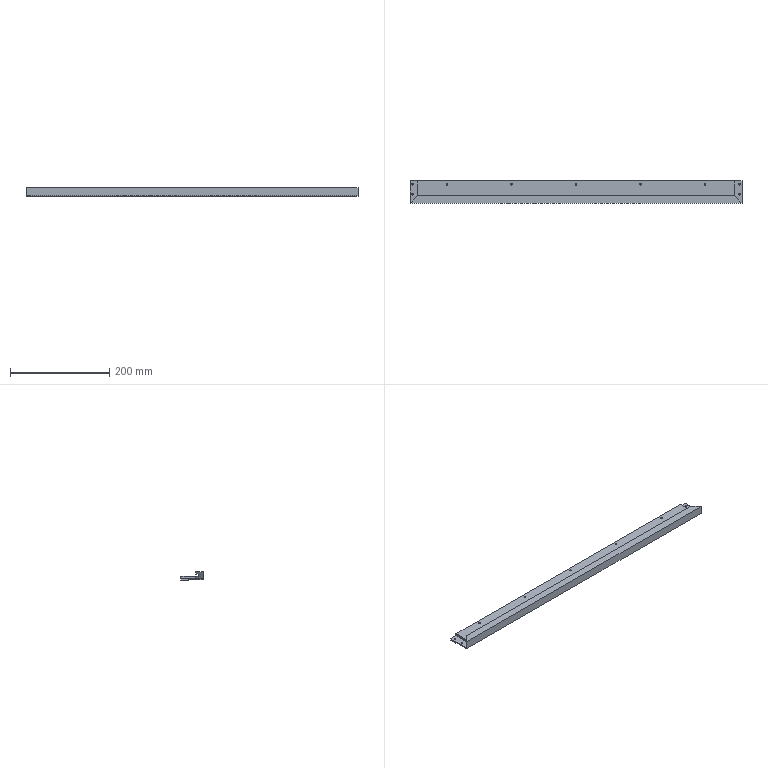Component | SolidWorks | AUTO-SpinDryWashing-01-03000004-1 | 1 solid | 36 faces | box 670 x 45 x 18 mm | volume 297172 mm3 | cylinder 18 | plane 18 | commonest cylinder face diameters 3.3 x18 | material AISI 316 Stainless Steel Sheet (SS)
build123d program:
from build123d import *

# Parameters (mm, degrees)
SKETCH1_W           = 20
SKETCH1_H           = 15
BOSS_EXTRUDE1_DEPTH = 335
SKETCH2_W           = 15
SKETCH2_H           = 30
BOSS_EXTRUDE2_DEPTH = 335
CUT_EXTRUDE2_DEPTH  = 671.746
CUT_EXTRUDE3_DEPTH  = 13
M4_TAPPED_HOLE1_D   = 3.3
M4_TAPPED_HOLE2_D   = 3.3
BOSS_EXTRUDE3_DEPTH = 2
SKETCH11_W          = 4
SKETCH11_H          = 15
CUT_EXTRUDE4_DEPTH  = 671.779


with BuildPart() as part:
    # Sketch1 → Boss-Extrude1 (new, symmetric)
    with BuildSketch(Plane.XY):
        with Locations((0, 7.5)):
            Rectangle(SKETCH1_W, SKETCH1_H)
    extrude(amount=BOSS_EXTRUDE1_DEPTH, both=True)

    # Sketch2 → Boss-Extrude2 (add, symmetric)
    with BuildSketch(Plane.XY):
        with Locations((-2.5, -15)):
            Rectangle(SKETCH2_W, SKETCH2_H)
    extrude(amount=BOSS_EXTRUDE2_DEPTH, both=True)

    # Sketch3 → Cut-Extrude2 (cut, through all)
    with BuildSketch(Plane.XY.offset(335)):
        Polygon((-10, 15), (-2, 15), (-2, -10), (-2, -20), (-7, -20), (-7, -15), (-10, -15), align=None)
    extrude(amount=-CUT_EXTRUDE2_DEPTH, mode=Mode.SUBTRACT)

    # Sketch4 → Cut-Extrude3 (cut)
    with BuildSketch(Plane.ZY.offset(10)):
        Polygon((-335, -30), (-335, -15), (-335, 15), (-320, 15), (-320, -15), align=None)
    cut_extrude3 = extrude(amount=-CUT_EXTRUDE3_DEPTH, mode=Mode.SUBTRACT)

    # Mirror1: Cut-Extrude3 across plane
    add(cut_extrude3.mirror(Plane.XY), mode=Mode.SUBTRACT)

    # M4 Tapped Hole1 (through all)
    with Locations(Plane(origin=(10, 0, 0), x_dir=(0, 0, -1), z_dir=(1, 0, 0))):
        with Locations((0, 8), (-130, 8), (-260, 8), (130, 8), (260, 8)):
            Hole(M4_TAPPED_HOLE1_D / 2)

    # M4 Tapped Hole2 (through all)
    with Locations(Plane.ZY.offset(-3)):
        with Locations((-330, -12), (-330, 8), (330, 8), (330, -12)):
            Hole(M4_TAPPED_HOLE2_D / 2)

    # Sketch10 → Boss-Extrude3 (add)
    with BuildSketch(Plane.ZY.offset(10)):
        Polygon((335, -30), (320, -15), (-320, -15), (-335, -30), align=None)
    extrude(amount=BOSS_EXTRUDE3_DEPTH)

    # Sketch11 → Cut-Extrude4 (cut, through all)
    with BuildSketch(Plane.XY.offset(335)):
        with Locations((8, 7.5)):
            Rectangle(SKETCH11_W, SKETCH11_H)
    extrude(amount=-CUT_EXTRUDE4_DEPTH, mode=Mode.SUBTRACT)


solid = part.part

# Placed as in the assembly
solid = solid.moved(Location((0, 408, 53), (0, 90, 0)))